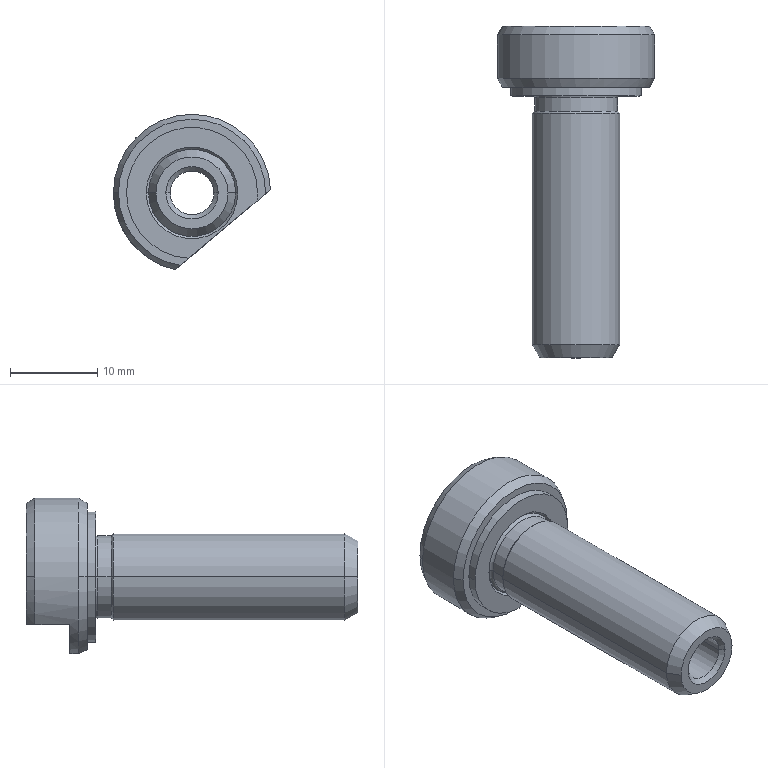Component | SolidWorks | JB_T8045.3-1999QuickChangeDrillBushing10_5_30-1 | 1 solid | 35 faces | box 17.99 x 38 x 17.79 mm | volume 3154 mm3 | cone 16 | cylinder 10 | plane 7 | torus 2 | commonest cylinder face diameters 15 x3 5 x2 10 x2 9.5 x2 18 x1 | material Nickel
STEP:
#1=COLOUR_RGB('',0.7922,0.8196,0.9333);
#2=FILL_AREA_STYLE_COLOUR('',#1);
#3=FILL_AREA_STYLE('',(#2));
#4=SURFACE_STYLE_FILL_AREA(#3);
#5=SURFACE_SIDE_STYLE('',(#4));
#6=SURFACE_STYLE_USAGE(.BOTH.,#5);
#7=PRESENTATION_STYLE_ASSIGNMENT((#6));
#8=CARTESIAN_POINT('',(-0.1628,10.827,2.067));
#9=VERTEX_POINT('',#8);
#10=CARTESIAN_POINT('',(0.1628,10.827,2.067));
#11=VERTEX_POINT('',#10);
#12=CARTESIAN_POINT('',(0.,10.827,2.067));
#13=DIRECTION('',(0.,-1.,0.));
#14=DIRECTION('',(1.,0.,0.));
#15=AXIS2_PLACEMENT_3D('',#12,#13,#14);
#16=CIRCLE('',#15,0.1628);
#17=EDGE_CURVE('',#9,#11,#16,.T.);
#18=ORIENTED_EDGE('',*,*,#17,.F.);
#19=CARTESIAN_POINT('',(-0.1969,10.886,2.067));
#20=VERTEX_POINT('',#19);
#21=CARTESIAN_POINT('',(-0.1969,10.886,2.067));
#22=DIRECTION('',(-0.5,0.866,-0.));
#23=VECTOR('',#22,39.37);
#24=LINE('',#21,#23);
#25=EDGE_CURVE('',#9,#20,#24,.T.);
#26=ORIENTED_EDGE('',*,*,#25,.T.);
#27=CARTESIAN_POINT('',(0.1969,10.886,2.067));
#28=VERTEX_POINT('',#27);
#29=CARTESIAN_POINT('',(0.,10.886,2.067));
#30=DIRECTION('',(0.,1.,0.));
#31=DIRECTION('',(1.,0.,0.));
#32=AXIS2_PLACEMENT_3D('',#29,#30,#31);
#33=CIRCLE('',#32,0.1969);
#34=EDGE_CURVE('',#28,#20,#33,.T.);
#35=ORIENTED_EDGE('',*,*,#34,.F.);
#36=CARTESIAN_POINT('',(0.1969,10.886,2.067));
#37=DIRECTION('',(0.5,0.866,0.));
#38=VECTOR('',#37,39.37);
#39=LINE('',#36,#38);
#40=EDGE_CURVE('',#11,#28,#39,.T.);
#41=ORIENTED_EDGE('',*,*,#40,.F.);
#42=EDGE_LOOP('',(#18,#26,#35,#41));
#43=FACE_OUTER_BOUND('',#42,.T.);
#44=CARTESIAN_POINT('',(0.,10.886,2.067));
#45=DIRECTION('',(0.,1.,0.));
#46=DIRECTION('',(1.,0.,0.));
#47=AXIS2_PLACEMENT_3D('',#44,#45,#46);
#48=CONICAL_SURFACE('',#47,0.1969,0.5236);
#49=ADVANCED_FACE('',(#43),#48,.T.);
#50=CARTESIAN_POINT('',(-0.1969,12.018,2.067));
#51=VERTEX_POINT('',#50);
#52=CARTESIAN_POINT('',(0.1969,12.018,2.067));
#53=VERTEX_POINT('',#52);
#54=CARTESIAN_POINT('',(0.,12.018,2.067));
#55=DIRECTION('',(0.,1.,0.));
#56=DIRECTION('',(1.,0.,0.));
#57=AXIS2_PLACEMENT_3D('',#54,#55,#56);
#58=CIRCLE('',#57,0.1969);
#59=EDGE_CURVE('',#51,#53,#58,.T.);
#60=ORIENTED_EDGE('',*,*,#59,.F.);
#61=CARTESIAN_POINT('',(-0.187,12.001,2.067));
#62=VERTEX_POINT('',#61);
#63=CARTESIAN_POINT('',(-0.2067,12.001,2.067));
#64=DIRECTION('',(0.,0.,-1.));
#65=DIRECTION('',(-1.,0.,0.));
#66=AXIS2_PLACEMENT_3D('',#63,#64,#65);
#67=CIRCLE('',#66,0.01969);
#68=EDGE_CURVE('',#51,#62,#67,.T.);
#69=ORIENTED_EDGE('',*,*,#68,.T.);
#70=CARTESIAN_POINT('',(0.187,12.001,2.067));
#71=VERTEX_POINT('',#70);
#72=CARTESIAN_POINT('',(0.,12.001,2.067));
#73=DIRECTION('',(0.,-1.,0.));
#74=DIRECTION('',(1.,0.,0.));
#75=AXIS2_PLACEMENT_3D('',#72,#73,#74);
#76=CIRCLE('',#75,0.187);
#77=EDGE_CURVE('',#71,#62,#76,.T.);
#78=ORIENTED_EDGE('',*,*,#77,.F.);
#79=CARTESIAN_POINT('',(0.2067,12.001,2.067));
#80=DIRECTION('',(-0.,0.,1.));
#81=DIRECTION('',(1.,0.,0.));
#82=AXIS2_PLACEMENT_3D('',#79,#80,#81);
#83=CIRCLE('',#82,0.01969);
#84=EDGE_CURVE('',#53,#71,#83,.T.);
#85=ORIENTED_EDGE('',*,*,#84,.F.);
#86=EDGE_LOOP('',(#60,#69,#78,#85));
#87=FACE_OUTER_BOUND('',#86,.T.);
#88=CARTESIAN_POINT('',(0.,12.001,2.067));
#89=DIRECTION('',(0.,1.,0.));
#90=DIRECTION('',(1.,0.,0.));
#91=AXIS2_PLACEMENT_3D('',#88,#89,#90);
#92=TOROIDAL_SURFACE('',#91,0.2067,0.01969);
#93=ADVANCED_FACE('',(#87),#92,.F.);
#94=ORIENTED_EDGE('',*,*,#59,.T.);
#95=CARTESIAN_POINT('',(0.2067,12.008,2.067));
#96=VERTEX_POINT('',#95);
#97=CARTESIAN_POINT('',(0.2067,12.008,2.067));
#98=DIRECTION('',(0.7071,-0.7071,0.));
#99=VECTOR('',#98,39.37);
#100=LINE('',#97,#99);
#101=EDGE_CURVE('',#53,#96,#100,.T.);
#102=ORIENTED_EDGE('',*,*,#101,.T.);
#103=CARTESIAN_POINT('',(-0.2067,12.008,2.067));
#104=VERTEX_POINT('',#103);
#105=CARTESIAN_POINT('',(0.,12.008,2.067));
#106=DIRECTION('',(0.,1.,0.));
#107=DIRECTION('',(1.,0.,0.));
#108=AXIS2_PLACEMENT_3D('',#105,#106,#107);
#109=CIRCLE('',#108,0.2067);
#110=EDGE_CURVE('',#104,#96,#109,.T.);
#111=ORIENTED_EDGE('',*,*,#110,.F.);
#112=CARTESIAN_POINT('',(-0.2067,12.008,2.067));
#113=DIRECTION('',(-0.7071,-0.7071,-0.));
#114=VECTOR('',#113,39.37);
#115=LINE('',#112,#114);
#116=EDGE_CURVE('',#51,#104,#115,.T.);
#117=ORIENTED_EDGE('',*,*,#116,.F.);
#118=EDGE_LOOP('',(#94,#102,#111,#117));
#119=FACE_OUTER_BOUND('',#118,.T.);
#120=CARTESIAN_POINT('',(0.,12.008,2.067));
#121=DIRECTION('',(0.,-1.,0.));
#122=DIRECTION('',(-1.,0.,0.));
#123=AXIS2_PLACEMENT_3D('',#120,#121,#122);
#124=CONICAL_SURFACE('',#123,0.2067,0.7854);
#125=ADVANCED_FACE('',(#119),#124,.F.);
#126=CARTESIAN_POINT('',(0.187,11.939,2.067));
#127=VERTEX_POINT('',#126);
#128=CARTESIAN_POINT('',(-0.187,11.939,2.067));
#129=VERTEX_POINT('',#128);
#130=CARTESIAN_POINT('',(0.,11.939,2.067));
#131=DIRECTION('',(0.,1.,0.));
#132=DIRECTION('',(1.,0.,0.));
#133=AXIS2_PLACEMENT_3D('',#130,#131,#132);
#134=CIRCLE('',#133,0.187);
#135=EDGE_CURVE('',#127,#129,#134,.T.);
#136=ORIENTED_EDGE('',*,*,#135,.F.);
#137=CARTESIAN_POINT('',(0.1969,11.929,2.067));
#138=VERTEX_POINT('',#137);
#139=CARTESIAN_POINT('',(0.187,11.939,2.067));
#140=DIRECTION('',(0.7071,-0.7071,0.));
#141=VECTOR('',#140,39.37);
#142=LINE('',#139,#141);
#143=EDGE_CURVE('',#127,#138,#142,.T.);
#144=ORIENTED_EDGE('',*,*,#143,.T.);
#145=CARTESIAN_POINT('',(-0.1969,11.929,2.067));
#146=VERTEX_POINT('',#145);
#147=CARTESIAN_POINT('',(0.,11.929,2.067));
#148=DIRECTION('',(0.,-1.,0.));
#149=DIRECTION('',(-1.,0.,0.));
#150=AXIS2_PLACEMENT_3D('',#147,#148,#149);
#151=CIRCLE('',#150,0.1969);
#152=EDGE_CURVE('',#146,#138,#151,.T.);
#153=ORIENTED_EDGE('',*,*,#152,.F.);
#154=CARTESIAN_POINT('',(-0.187,11.939,2.067));
#155=DIRECTION('',(-0.7071,-0.7071,-0.));
#156=VECTOR('',#155,39.37);
#157=LINE('',#154,#156);
#158=EDGE_CURVE('',#129,#146,#157,.T.);
#159=ORIENTED_EDGE('',*,*,#158,.F.);
#160=EDGE_LOOP('',(#136,#144,#153,#159));
#161=FACE_OUTER_BOUND('',#160,.T.);
#162=CARTESIAN_POINT('',(0.,11.939,2.067));
#163=DIRECTION('',(0.,-1.,0.));
#164=DIRECTION('',(-1.,0.,0.));
#165=AXIS2_PLACEMENT_3D('',#162,#163,#164);
#166=CONICAL_SURFACE('',#165,0.187,0.7854);
#167=ADVANCED_FACE('',(#161),#166,.T.);
#168=CARTESIAN_POINT('',(0.09843,10.846,2.067));
#169=VERTEX_POINT('',#168);
#170=CARTESIAN_POINT('',(-0.09843,10.846,2.067));
#171=VERTEX_POINT('',#170);
#172=CARTESIAN_POINT('',(0.,10.846,2.067));
#173=DIRECTION('',(0.,-1.,0.));
#174=DIRECTION('',(1.,0.,0.));
#175=AXIS2_PLACEMENT_3D('',#172,#173,#174);
#176=CIRCLE('',#175,0.09843);
#177=EDGE_CURVE('',#169,#171,#176,.T.);
#178=ORIENTED_EDGE('',*,*,#177,.F.);
#179=CARTESIAN_POINT('',(0.1181,10.827,2.067));
#180=VERTEX_POINT('',#179);
#181=CARTESIAN_POINT('',(0.1181,10.827,2.067));
#182=DIRECTION('',(0.7071,-0.7071,0.));
#183=VECTOR('',#182,39.37);
#184=LINE('',#181,#183);
#185=EDGE_CURVE('',#169,#180,#184,.T.);
#186=ORIENTED_EDGE('',*,*,#185,.T.);
#187=CARTESIAN_POINT('',(-0.1181,10.827,2.067));
#188=VERTEX_POINT('',#187);
#189=CARTESIAN_POINT('',(0.,10.827,2.067));
#190=DIRECTION('',(0.,1.,0.));
#191=DIRECTION('',(1.,0.,0.));
#192=AXIS2_PLACEMENT_3D('',#189,#190,#191);
#193=CIRCLE('',#192,0.1181);
#194=EDGE_CURVE('',#188,#180,#193,.T.);
#195=ORIENTED_EDGE('',*,*,#194,.F.);
#196=CARTESIAN_POINT('',(-0.1181,10.827,2.067));
#197=DIRECTION('',(-0.7071,-0.7071,-0.));
#198=VECTOR('',#197,39.37);
#199=LINE('',#196,#198);
#200=EDGE_CURVE('',#171,#188,#199,.T.);
#201=ORIENTED_EDGE('',*,*,#200,.F.);
#202=EDGE_LOOP('',(#178,#186,#195,#201));
#203=FACE_OUTER_BOUND('',#202,.T.);
#204=CARTESIAN_POINT('',(0.,10.827,2.067));
#205=DIRECTION('',(0.,-1.,0.));
#206=DIRECTION('',(-1.,0.,0.));
#207=AXIS2_PLACEMENT_3D('',#204,#205,#206);
#208=CONICAL_SURFACE('',#207,0.1181,0.7854);
#209=ADVANCED_FACE('',(#203),#208,.F.);
#210=CARTESIAN_POINT('',(-0.09843,12.264,2.067));
#211=VERTEX_POINT('',#210);
#212=CARTESIAN_POINT('',(0.09843,12.264,2.067));
#213=VERTEX_POINT('',#212);
#214=CARTESIAN_POINT('',(0.,12.264,2.067));
#215=DIRECTION('',(0.,1.,0.));
#216=DIRECTION('',(-1.,0.,0.));
#217=AXIS2_PLACEMENT_3D('',#214,#215,#216);
#218=CIRCLE('',#217,0.09843);
#219=EDGE_CURVE('',#211,#213,#218,.T.);
#220=ORIENTED_EDGE('',*,*,#219,.F.);
#221=CARTESIAN_POINT('',(-0.1325,12.323,2.067));
#222=VERTEX_POINT('',#221);
#223=CARTESIAN_POINT('',(-0.09843,12.264,2.067));
#224=DIRECTION('',(-0.5,0.866,-0.));
#225=VECTOR('',#224,39.37);
#226=LINE('',#223,#225);
#227=EDGE_CURVE('',#211,#222,#226,.T.);
#228=ORIENTED_EDGE('',*,*,#227,.T.);
#229=CARTESIAN_POINT('',(0.1325,12.323,2.067));
#230=VERTEX_POINT('',#229);
#231=CARTESIAN_POINT('',(0.,12.323,2.067));
#232=DIRECTION('',(0.,-1.,0.));
#233=DIRECTION('',(-1.,0.,0.));
#234=AXIS2_PLACEMENT_3D('',#231,#232,#233);
#235=CIRCLE('',#234,0.1325);
#236=EDGE_CURVE('',#230,#222,#235,.T.);
#237=ORIENTED_EDGE('',*,*,#236,.F.);
#238=CARTESIAN_POINT('',(0.09843,12.264,2.067));
#239=DIRECTION('',(0.5,0.866,0.));
#240=VECTOR('',#239,39.37);
#241=LINE('',#238,#240);
#242=EDGE_CURVE('',#213,#230,#241,.T.);
#243=ORIENTED_EDGE('',*,*,#242,.F.);
#244=EDGE_LOOP('',(#220,#228,#237,#243));
#245=FACE_OUTER_BOUND('',#244,.T.);
#246=CARTESIAN_POINT('',(0.,12.264,2.067));
#247=DIRECTION('',(0.,1.,0.));
#248=DIRECTION('',(1.,0.,0.));
#249=AXIS2_PLACEMENT_3D('',#246,#247,#248);
#250=CONICAL_SURFACE('',#249,0.09843,0.5236);
#251=ADVANCED_FACE('',(#245),#250,.F.);
#252=ORIENTED_EDGE('',*,*,#177,.T.);
#253=CARTESIAN_POINT('',(-0.09843,16.352,2.067));
#254=DIRECTION('',(0.,1.,0.));
#255=VECTOR('',#254,39.37);
#256=LINE('',#253,#255);
#257=EDGE_CURVE('',#171,#211,#256,.T.);
#258=ORIENTED_EDGE('',*,*,#257,.T.);
#259=ORIENTED_EDGE('',*,*,#219,.T.);
#260=CARTESIAN_POINT('',(0.09843,16.352,2.067));
#261=DIRECTION('',(0.,1.,0.));
#262=VECTOR('',#261,39.37);
#263=LINE('',#260,#262);
#264=EDGE_CURVE('',#169,#213,#263,.T.);
#265=ORIENTED_EDGE('',*,*,#264,.F.);
#266=EDGE_LOOP('',(#252,#258,#259,#265));
#267=FACE_OUTER_BOUND('',#266,.T.);
#268=CARTESIAN_POINT('',(0.,16.352,2.067));
#269=DIRECTION('',(0.,1.,0.));
#270=DIRECTION('',(1.,0.,0.));
#271=AXIS2_PLACEMENT_3D('',#268,#269,#270);
#272=CYLINDRICAL_SURFACE('',#271,0.09843);
#273=ADVANCED_FACE('',(#267),#272,.F.);
#274=ORIENTED_EDGE('',*,*,#34,.T.);
#275=CARTESIAN_POINT('',(-0.1969,16.352,2.067));
#276=DIRECTION('',(0.,1.,0.));
#277=VECTOR('',#276,39.37);
#278=LINE('',#275,#277);
#279=EDGE_CURVE('',#20,#146,#278,.T.);
#280=ORIENTED_EDGE('',*,*,#279,.T.);
#281=ORIENTED_EDGE('',*,*,#152,.T.);
#282=CARTESIAN_POINT('',(0.1969,16.352,2.067));
#283=DIRECTION('',(0.,1.,0.));
#284=VECTOR('',#283,39.37);
#285=LINE('',#282,#284);
#286=EDGE_CURVE('',#28,#138,#285,.T.);
#287=ORIENTED_EDGE('',*,*,#286,.F.);
#288=EDGE_LOOP('',(#274,#280,#281,#287));
#289=FACE_OUTER_BOUND('',#288,.T.);
#290=CARTESIAN_POINT('',(0.,16.352,2.067));
#291=DIRECTION('',(0.,1.,0.));
#292=DIRECTION('',(1.,0.,0.));
#293=AXIS2_PLACEMENT_3D('',#290,#291,#292);
#294=CYLINDRICAL_SURFACE('',#293,0.1969);
#295=ADVANCED_FACE('',(#289),#294,.T.);
#296=ORIENTED_EDGE('',*,*,#135,.T.);
#297=CARTESIAN_POINT('',(-0.187,16.352,2.067));
#298=DIRECTION('',(0.,1.,0.));
#299=VECTOR('',#298,39.37);
#300=LINE('',#297,#299);
#301=EDGE_CURVE('',#129,#62,#300,.T.);
#302=ORIENTED_EDGE('',*,*,#301,.T.);
#303=CARTESIAN_POINT('',(0.,12.001,2.067));
#304=DIRECTION('',(0.,-1.,0.));
#305=DIRECTION('',(1.,0.,0.));
#306=AXIS2_PLACEMENT_3D('',#303,#304,#305);
#307=CIRCLE('',#306,0.187);
#308=EDGE_CURVE('',#62,#71,#307,.T.);
#309=ORIENTED_EDGE('',*,*,#308,.T.);
#310=CARTESIAN_POINT('',(0.187,16.352,2.067));
#311=DIRECTION('',(0.,1.,0.));
#312=VECTOR('',#311,39.37);
#313=LINE('',#310,#312);
#314=EDGE_CURVE('',#127,#71,#313,.T.);
#315=ORIENTED_EDGE('',*,*,#314,.F.);
#316=EDGE_LOOP('',(#296,#302,#309,#315));
#317=FACE_OUTER_BOUND('',#316,.T.);
#318=CARTESIAN_POINT('',(0.,16.352,2.067));
#319=DIRECTION('',(0.,1.,0.));
#320=DIRECTION('',(1.,0.,0.));
#321=AXIS2_PLACEMENT_3D('',#318,#319,#320);
#322=CYLINDRICAL_SURFACE('',#321,0.187);
#323=ADVANCED_FACE('',(#317),#322,.T.);
#324=CARTESIAN_POINT('',(-0.3316,12.047,2.067));
#325=VERTEX_POINT('',#324);
#326=CARTESIAN_POINT('',(-0.0532,12.047,1.74));
#327=VERTEX_POINT('',#326);
#328=CARTESIAN_POINT('',(0.,12.047,2.067));
#329=DIRECTION('',(0.,-1.,0.));
#330=DIRECTION('',(1.,0.,-0.));
#331=AXIS2_PLACEMENT_3D('',#328,#329,#330);
#332=CIRCLE('',#331,0.3316);
#333=EDGE_CURVE('',#325,#327,#332,.T.);
#334=ORIENTED_EDGE('',*,*,#333,.F.);
#335=CARTESIAN_POINT('',(-0.3543,12.087,2.067));
#336=VERTEX_POINT('',#335);
#337=CARTESIAN_POINT('',(-0.3543,12.087,2.067));
#338=DIRECTION('',(-0.5,0.866,-0.));
#339=VECTOR('',#338,39.37);
#340=LINE('',#337,#339);
#341=EDGE_CURVE('',#325,#336,#340,.T.);
#342=ORIENTED_EDGE('',*,*,#341,.T.);
#343=CARTESIAN_POINT('',(-0.07566,12.087,1.721));
#344=VERTEX_POINT('',#343);
#345=CARTESIAN_POINT('',(0.,12.087,2.067));
#346=DIRECTION('',(0.,1.,0.));
#347=DIRECTION('',(1.,0.,0.));
#348=AXIS2_PLACEMENT_3D('',#345,#346,#347);
#349=CIRCLE('',#348,0.3543);
#350=EDGE_CURVE('',#344,#336,#349,.T.);
#351=ORIENTED_EDGE('',*,*,#350,.F.);
#352=CARTESIAN_POINT('',(-0.07566,12.087,1.721));
#353=CARTESIAN_POINT('',(-0.06828,12.073,1.727));
#354=CARTESIAN_POINT('',(-0.0608,12.06,1.733));
#355=CARTESIAN_POINT('',(-0.0532,12.047,1.74));
#356=B_SPLINE_CURVE_WITH_KNOTS('',3,(#352,#353,#354,#355),.UNSPECIFIED.,.F.,.F.,(4,4),(0.01817,0.01941),.UNSPECIFIED.);
#357=EDGE_CURVE('',#344,#327,#356,.T.);
#358=ORIENTED_EDGE('',*,*,#357,.T.);
#359=EDGE_LOOP('',(#334,#342,#351,#358));
#360=FACE_OUTER_BOUND('',#359,.T.);
#361=CARTESIAN_POINT('',(0.,12.087,2.067));
#362=DIRECTION('',(0.,1.,0.));
#363=DIRECTION('',(1.,0.,0.));
#364=AXIS2_PLACEMENT_3D('',#361,#362,#363);
#365=CONICAL_SURFACE('',#364,0.3543,0.5236);
#366=ADVANCED_FACE('',(#360),#365,.T.);
#367=ORIENTED_EDGE('',*,*,#341,.F.);
#368=CARTESIAN_POINT('',(0.3316,12.047,2.067));
#369=VERTEX_POINT('',#368);
#370=CARTESIAN_POINT('',(0.,12.047,2.067));
#371=DIRECTION('',(0.,-1.,0.));
#372=DIRECTION('',(1.,0.,0.));
#373=AXIS2_PLACEMENT_3D('',#370,#371,#372);
#374=CIRCLE('',#373,0.3316);
#375=EDGE_CURVE('',#369,#325,#374,.T.);
#376=ORIENTED_EDGE('',*,*,#375,.F.);
#377=CARTESIAN_POINT('',(0.3369,12.056,2.067));
#378=VERTEX_POINT('',#377);
#379=CARTESIAN_POINT('',(0.3543,12.087,2.067));
#380=DIRECTION('',(0.5,0.866,0.));
#381=VECTOR('',#380,39.37);
#382=LINE('',#379,#381);
#383=EDGE_CURVE('',#369,#378,#382,.T.);
#384=ORIENTED_EDGE('',*,*,#383,.T.);
#385=CARTESIAN_POINT('',(0.354,12.087,2.081));
#386=VERTEX_POINT('',#385);
#387=CARTESIAN_POINT('',(0.3369,12.056,2.067));
#388=CARTESIAN_POINT('',(0.3427,12.066,2.072));
#389=CARTESIAN_POINT('',(0.3484,12.076,2.077));
#390=CARTESIAN_POINT('',(0.354,12.087,2.081));
#391=B_SPLINE_CURVE_WITH_KNOTS('',3,(#387,#388,#389,#390),.UNSPECIFIED.,.F.,.F.,(4,4),(0.03623,0.03717),.UNSPECIFIED.);
#392=EDGE_CURVE('',#378,#386,#391,.T.);
#393=ORIENTED_EDGE('',*,*,#392,.T.);
#394=CARTESIAN_POINT('',(0.,12.087,2.067));
#395=DIRECTION('',(0.,1.,0.));
#396=DIRECTION('',(1.,0.,0.));
#397=AXIS2_PLACEMENT_3D('',#394,#395,#396);
#398=CIRCLE('',#397,0.3543);
#399=EDGE_CURVE('',#336,#386,#398,.T.);
#400=ORIENTED_EDGE('',*,*,#399,.F.);
#401=EDGE_LOOP('',(#367,#376,#384,#393,#400));
#402=FACE_OUTER_BOUND('',#401,.T.);
#403=CARTESIAN_POINT('',(0.,12.087,2.067));
#404=DIRECTION('',(0.,1.,0.));
#405=DIRECTION('',(1.,0.,0.));
#406=AXIS2_PLACEMENT_3D('',#403,#404,#405);
#407=CONICAL_SURFACE('',#406,0.3543,0.5236);
#408=ADVANCED_FACE('',(#402),#407,.T.);
#409=CARTESIAN_POINT('',(-0.01459,12.008,1.772));
#410=VERTEX_POINT('',#409);
#411=CARTESIAN_POINT('',(-0.2953,12.008,2.067));
#412=VERTEX_POINT('',#411);
#413=CARTESIAN_POINT('',(0.,12.008,2.067));
#414=DIRECTION('',(0.,1.,0.));
#415=DIRECTION('',(1.,0.,0.));
#416=AXIS2_PLACEMENT_3D('',#413,#414,#415);
#417=CIRCLE('',#416,0.2953);
#418=EDGE_CURVE('',#410,#412,#417,.T.);
#419=ORIENTED_EDGE('',*,*,#418,.T.);
#420=CARTESIAN_POINT('',(-0.2953,12.047,2.067));
#421=VERTEX_POINT('',#420);
#422=CARTESIAN_POINT('',(-0.2953,16.352,2.067));
#423=DIRECTION('',(0.,1.,0.));
#424=VECTOR('',#423,39.37);
#425=LINE('',#422,#424);
#426=EDGE_CURVE('',#412,#421,#425,.T.);
#427=ORIENTED_EDGE('',*,*,#426,.T.);
#428=CARTESIAN_POINT('',(-0.01459,12.047,1.772));
#429=VERTEX_POINT('',#428);
#430=CARTESIAN_POINT('',(0.,12.047,2.067));
#431=DIRECTION('',(0.,1.,0.));
#432=DIRECTION('',(1.,0.,0.));
#433=AXIS2_PLACEMENT_3D('',#430,#431,#432);
#434=CIRCLE('',#433,0.2953);
#435=EDGE_CURVE('',#429,#421,#434,.T.);
#436=ORIENTED_EDGE('',*,*,#435,.F.);
#437=CARTESIAN_POINT('',(-0.01459,16.352,1.772));
#438=DIRECTION('',(0.,1.,0.));
#439=VECTOR('',#438,39.37);
#440=LINE('',#437,#439);
#441=EDGE_CURVE('',#410,#429,#440,.T.);
#442=ORIENTED_EDGE('',*,*,#441,.F.);
#443=EDGE_LOOP('',(#419,#427,#436,#442));
#444=FACE_OUTER_BOUND('',#443,.T.);
#445=CARTESIAN_POINT('',(0.,16.352,2.067));
#446=DIRECTION('',(0.,1.,0.));
#447=DIRECTION('',(1.,0.,0.));
#448=AXIS2_PLACEMENT_3D('',#445,#446,#447);
#449=CYLINDRICAL_SURFACE('',#448,0.2953);
#450=ADVANCED_FACE('',(#444),#449,.T.);
#451=ORIENTED_EDGE('',*,*,#426,.F.);
#452=CARTESIAN_POINT('',(0.2953,12.008,2.067));
#453=VERTEX_POINT('',#452);
#454=CARTESIAN_POINT('',(0.,12.008,2.067));
#455=DIRECTION('',(0.,1.,0.));
#456=DIRECTION('',(1.,0.,0.));
#457=AXIS2_PLACEMENT_3D('',#454,#455,#456);
#458=CIRCLE('',#457,0.2953);
#459=EDGE_CURVE('',#412,#453,#458,.T.);
#460=ORIENTED_EDGE('',*,*,#459,.T.);
#461=CARTESIAN_POINT('',(0.2953,12.047,2.067));
#462=VERTEX_POINT('',#461);
#463=CARTESIAN_POINT('',(0.2953,16.352,2.067));
#464=DIRECTION('',(0.,1.,0.));
#465=VECTOR('',#464,39.37);
#466=LINE('',#463,#465);
#467=EDGE_CURVE('',#453,#462,#466,.T.);
#468=ORIENTED_EDGE('',*,*,#467,.T.);
#469=CARTESIAN_POINT('',(0.,12.047,2.067));
#470=DIRECTION('',(0.,1.,0.));
#471=DIRECTION('',(1.,0.,0.));
#472=AXIS2_PLACEMENT_3D('',#469,#470,#471);
#473=CIRCLE('',#472,0.2953);
#474=EDGE_CURVE('',#421,#462,#473,.T.);
#475=ORIENTED_EDGE('',*,*,#474,.F.);
#476=EDGE_LOOP('',(#451,#460,#468,#475));
#477=FACE_OUTER_BOUND('',#476,.T.);
#478=CARTESIAN_POINT('',(0.,16.352,2.067));
#479=DIRECTION('',(0.,1.,0.));
#480=DIRECTION('',(1.,0.,0.));
#481=AXIS2_PLACEMENT_3D('',#478,#479,#480);
#482=CYLINDRICAL_SURFACE('',#481,0.2953);
#483=ADVANCED_FACE('',(#477),#482,.T.);
#484=CARTESIAN_POINT('',(0.3316,12.323,2.067));
#485=VERTEX_POINT('',#484);
#486=CARTESIAN_POINT('',(0.3316,12.323,2.062));
#487=VERTEX_POINT('',#486);
#488=CARTESIAN_POINT('',(0.,12.323,2.067));
#489=DIRECTION('',(0.,1.,0.));
#490=DIRECTION('',(-1.,0.,0.));
#491=AXIS2_PLACEMENT_3D('',#488,#489,#490);
#492=CIRCLE('',#491,0.3316);
#493=EDGE_CURVE('',#485,#487,#492,.T.);
#494=ORIENTED_EDGE('',*,*,#493,.F.);
#495=CARTESIAN_POINT('',(0.3369,12.314,2.067));
#496=VERTEX_POINT('',#495);
#497=CARTESIAN_POINT('',(0.3316,12.323,2.067));
#498=DIRECTION('',(0.5,-0.866,0.));
#499=VECTOR('',#498,39.37);
#500=LINE('',#497,#499);
#501=EDGE_CURVE('',#485,#496,#500,.T.);
#502=ORIENTED_EDGE('',*,*,#501,.T.);
#503=CARTESIAN_POINT('',(0.3369,12.314,2.067));
#504=CARTESIAN_POINT('',(0.3351,12.317,2.065));
#505=CARTESIAN_POINT('',(0.3333,12.32,2.064));
#506=CARTESIAN_POINT('',(0.3316,12.323,2.062));
#507=B_SPLINE_CURVE_WITH_KNOTS('',3,(#503,#504,#505,#506),.UNSPECIFIED.,.F.,.F.,(4,4),(0.01747,0.01777),.UNSPECIFIED.);
#508=EDGE_CURVE('',#496,#487,#507,.T.);
#509=ORIENTED_EDGE('',*,*,#508,.T.);
#510=EDGE_LOOP('',(#494,#502,#509));
#511=FACE_OUTER_BOUND('',#510,.T.);
#512=CARTESIAN_POINT('',(0.,12.323,2.067));
#513=DIRECTION('',(0.,-1.,0.));
#514=DIRECTION('',(-1.,0.,0.));
#515=AXIS2_PLACEMENT_3D('',#512,#513,#514);
#516=CONICAL_SURFACE('',#515,0.3316,0.5236);
#517=ADVANCED_FACE('',(#511),#516,.T.);
#518=ORIENTED_EDGE('',*,*,#501,.F.);
#519=CARTESIAN_POINT('',(-0.3316,12.323,2.067));
#520=VERTEX_POINT('',#519);
#521=CARTESIAN_POINT('',(0.,12.323,2.067));
#522=DIRECTION('',(0.,1.,0.));
#523=DIRECTION('',(-1.,0.,0.));
#524=AXIS2_PLACEMENT_3D('',#521,#522,#523);
#525=CIRCLE('',#524,0.3316);
#526=EDGE_CURVE('',#520,#485,#525,.T.);
#527=ORIENTED_EDGE('',*,*,#526,.F.);
#528=CARTESIAN_POINT('',(-0.3543,12.283,2.067));
#529=VERTEX_POINT('',#528);
#530=CARTESIAN_POINT('',(-0.3316,12.323,2.067));
#531=DIRECTION('',(-0.5,-0.866,-0.));
#532=VECTOR('',#531,39.37);
#533=LINE('',#530,#532);
#534=EDGE_CURVE('',#520,#529,#533,.T.);
#535=ORIENTED_EDGE('',*,*,#534,.T.);
#536=CARTESIAN_POINT('',(0.354,12.283,2.081));
#537=VERTEX_POINT('',#536);
#538=CARTESIAN_POINT('',(0.,12.283,2.067));
#539=DIRECTION('',(0.,-1.,0.));
#540=DIRECTION('',(-1.,0.,0.));
#541=AXIS2_PLACEMENT_3D('',#538,#539,#540);
#542=CIRCLE('',#541,0.3543);
#543=EDGE_CURVE('',#537,#529,#542,.T.);
#544=ORIENTED_EDGE('',*,*,#543,.F.);
#545=CARTESIAN_POINT('',(0.354,12.283,2.081));
#546=CARTESIAN_POINT('',(0.3484,12.294,2.077));
#547=CARTESIAN_POINT('',(0.3427,12.304,2.072));
#548=CARTESIAN_POINT('',(0.3369,12.314,2.067));
#549=B_SPLINE_CURVE_WITH_KNOTS('',3,(#545,#546,#547,#548),.UNSPECIFIED.,.F.,.F.,(4,4),(0.01652,0.01747),.UNSPECIFIED.);
#550=EDGE_CURVE('',#537,#496,#549,.T.);
#551=ORIENTED_EDGE('',*,*,#550,.T.);
#552=EDGE_LOOP('',(#518,#527,#535,#544,#551));
#553=FACE_OUTER_BOUND('',#552,.T.);
#554=CARTESIAN_POINT('',(0.,12.323,2.067));
#555=DIRECTION('',(0.,-1.,0.));
#556=DIRECTION('',(-1.,0.,0.));
#557=AXIS2_PLACEMENT_3D('',#554,#555,#556);
#558=CONICAL_SURFACE('',#557,0.3316,0.5236);
#559=ADVANCED_FACE('',(#553),#558,.T.);
#560=CARTESIAN_POINT('',(-0.07566,12.126,1.721));
#561=VERTEX_POINT('',#560);
#562=CARTESIAN_POINT('',(-0.07566,16.352,1.721));
#563=DIRECTION('',(0.,1.,0.));
#564=VECTOR('',#563,39.37);
#565=LINE('',#562,#564);
#566=EDGE_CURVE('',#344,#561,#565,.T.);
#567=ORIENTED_EDGE('',*,*,#566,.F.);
#568=ORIENTED_EDGE('',*,*,#350,.T.);
#569=ORIENTED_EDGE('',*,*,#399,.T.);
#570=CARTESIAN_POINT('',(0.354,16.352,2.081));
#571=DIRECTION('',(0.,-1.,0.));
#572=VECTOR('',#571,39.37);
#573=LINE('',#570,#572);
#574=EDGE_CURVE('',#537,#386,#573,.T.);
#575=ORIENTED_EDGE('',*,*,#574,.F.);
#576=ORIENTED_EDGE('',*,*,#543,.T.);
#577=CARTESIAN_POINT('',(-0.2805,12.283,1.85));
#578=VERTEX_POINT('',#577);
#579=CARTESIAN_POINT('',(0.,12.283,2.067));
#580=DIRECTION('',(0.,-1.,0.));
#581=DIRECTION('',(-1.,0.,0.));
#582=AXIS2_PLACEMENT_3D('',#579,#580,#581);
#583=CIRCLE('',#582,0.3543);
#584=EDGE_CURVE('',#529,#578,#583,.T.);
#585=ORIENTED_EDGE('',*,*,#584,.T.);
#586=CARTESIAN_POINT('',(-0.2805,12.126,1.85));
#587=VERTEX_POINT('',#586);
#588=CARTESIAN_POINT('',(-0.2805,16.352,1.85));
#589=DIRECTION('',(0.,1.,0.));
#590=VECTOR('',#589,39.37);
#591=LINE('',#588,#590);
#592=EDGE_CURVE('',#587,#578,#591,.T.);
#593=ORIENTED_EDGE('',*,*,#592,.F.);
#594=CARTESIAN_POINT('',(0.,12.126,2.067));
#595=DIRECTION('',(0.,1.,0.));
#596=DIRECTION('',(1.,0.,0.));
#597=AXIS2_PLACEMENT_3D('',#594,#595,#596);
#598=CIRCLE('',#597,0.3543);
#599=EDGE_CURVE('',#561,#587,#598,.T.);
#600=ORIENTED_EDGE('',*,*,#599,.F.);
#601=EDGE_LOOP('',(#567,#568,#569,#575,#576,#585,#593,#600));
#602=FACE_OUTER_BOUND('',#601,.T.);
#603=CARTESIAN_POINT('',(0.,16.352,2.067));
#604=DIRECTION('',(0.,1.,0.));
#605=DIRECTION('',(1.,0.,0.));
#606=AXIS2_PLACEMENT_3D('',#603,#604,#605);
#607=CYLINDRICAL_SURFACE('',#606,0.3543);
#608=ADVANCED_FACE('',(#602),#607,.T.);
#609=ORIENTED_EDGE('',*,*,#236,.T.);
#610=CARTESIAN_POINT('',(0.,12.323,2.067));
#611=DIRECTION('',(0.,-1.,0.));
#612=DIRECTION('',(-1.,0.,0.));
#613=AXIS2_PLACEMENT_3D('',#610,#611,#612);
#614=CIRCLE('',#613,0.1325);
#615=EDGE_CURVE('',#222,#230,#614,.T.);
#616=ORIENTED_EDGE('',*,*,#615,.T.);
#617=EDGE_LOOP('',(#609,#616));
#618=FACE_BOUND('',#617,.T.);
#619=CARTESIAN_POINT('',(0.07881,12.323,1.85));
#620=VERTEX_POINT('',#619);
#621=CARTESIAN_POINT('',(0.09072,12.323,1.86));
#622=DIRECTION('',(0.766,0.,0.6428));
#623=VECTOR('',#622,39.37);
#624=LINE('',#621,#623);
#625=EDGE_CURVE('',#620,#487,#624,.T.);
#626=ORIENTED_EDGE('',*,*,#625,.F.);
#627=CARTESIAN_POINT('',(-0.2511,12.323,1.85));
#628=VERTEX_POINT('',#627);
#629=CARTESIAN_POINT('',(0.,12.323,1.85));
#630=DIRECTION('',(1.,0.,0.));
#631=VECTOR('',#630,39.37);
#632=LINE('',#629,#631);
#633=EDGE_CURVE('',#628,#620,#632,.T.);
#634=ORIENTED_EDGE('',*,*,#633,.F.);
#635=CARTESIAN_POINT('',(0.,12.323,2.067));
#636=DIRECTION('',(0.,1.,0.));
#637=DIRECTION('',(-1.,0.,0.));
#638=AXIS2_PLACEMENT_3D('',#635,#636,#637);
#639=CIRCLE('',#638,0.3316);
#640=EDGE_CURVE('',#628,#520,#639,.T.);
#641=ORIENTED_EDGE('',*,*,#640,.T.);
#642=ORIENTED_EDGE('',*,*,#526,.T.);
#643=ORIENTED_EDGE('',*,*,#493,.T.);
#644=EDGE_LOOP('',(#626,#634,#641,#642,#643));
#645=FACE_OUTER_BOUND('',#644,.T.);
#646=CARTESIAN_POINT('',(0.,12.323,1.969));
#647=DIRECTION('',(0.,-1.,0.));
#648=DIRECTION('',(-1.,0.,-0.));
#649=AXIS2_PLACEMENT_3D('',#646,#647,#648);
#650=PLANE('',#649);
#651=ADVANCED_FACE('',(#618,#645),#650,.F.);
#652=ORIENTED_EDGE('',*,*,#534,.F.);
#653=ORIENTED_EDGE('',*,*,#640,.F.);
#654=CARTESIAN_POINT('',(-0.2511,12.323,1.85));
#655=CARTESIAN_POINT('',(-0.2611,12.31,1.85));
#656=CARTESIAN_POINT('',(-0.2708,12.297,1.85));
#657=CARTESIAN_POINT('',(-0.2805,12.283,1.85));
#658=B_SPLINE_CURVE_WITH_KNOTS('',3,(#654,#655,#656,#657),.UNSPECIFIED.,.F.,.F.,(4,4),(0.03099,0.03225),.UNSPECIFIED.);
#659=EDGE_CURVE('',#628,#578,#658,.T.);
#660=ORIENTED_EDGE('',*,*,#659,.T.);
#661=ORIENTED_EDGE('',*,*,#584,.F.);
#662=EDGE_LOOP('',(#652,#653,#660,#661));
#663=FACE_OUTER_BOUND('',#662,.T.);
#664=CARTESIAN_POINT('',(0.,12.323,2.067));
#665=DIRECTION('',(0.,-1.,0.));
#666=DIRECTION('',(-1.,0.,0.));
#667=AXIS2_PLACEMENT_3D('',#664,#665,#666);
#668=CONICAL_SURFACE('',#667,0.3316,0.5236);
#669=ADVANCED_FACE('',(#663),#668,.T.);
#670=CARTESIAN_POINT('',(0.3316,12.047,2.062));
#671=VERTEX_POINT('',#670);
#672=CARTESIAN_POINT('',(0.293,12.047,2.03));
#673=VERTEX_POINT('',#672);
#674=CARTESIAN_POINT('',(-0.03529,12.047,1.755));
#675=DIRECTION('',(-0.766,0.,-0.6428));
#676=VECTOR('',#675,39.37);
#677=LINE('',#674,#676);
#678=EDGE_CURVE('',#671,#673,#677,.T.);
#679=ORIENTED_EDGE('',*,*,#678,.F.);
#680=CARTESIAN_POINT('',(0.,12.047,2.067));
#681=DIRECTION('',(0.,-1.,0.));
#682=DIRECTION('',(1.,0.,0.));
#683=AXIS2_PLACEMENT_3D('',#680,#681,#682);
#684=CIRCLE('',#683,0.3316);
#685=EDGE_CURVE('',#671,#369,#684,.T.);
#686=ORIENTED_EDGE('',*,*,#685,.T.);
#687=ORIENTED_EDGE('',*,*,#375,.T.);
#688=ORIENTED_EDGE('',*,*,#333,.T.);
#689=CARTESIAN_POINT('',(-0.03529,12.047,1.755));
#690=DIRECTION('',(-0.766,0.,-0.6428));
#691=VECTOR('',#690,39.37);
#692=LINE('',#689,#691);
#693=EDGE_CURVE('',#429,#327,#692,.T.);
#694=ORIENTED_EDGE('',*,*,#693,.F.);
#695=ORIENTED_EDGE('',*,*,#435,.T.);
#696=ORIENTED_EDGE('',*,*,#474,.T.);
#697=CARTESIAN_POINT('',(0.,12.047,2.067));
#698=DIRECTION('',(0.,1.,0.));
#699=DIRECTION('',(1.,0.,0.));
#700=AXIS2_PLACEMENT_3D('',#697,#698,#699);
#701=CIRCLE('',#700,0.2953);
#702=EDGE_CURVE('',#462,#673,#701,.T.);
#703=ORIENTED_EDGE('',*,*,#702,.T.);
#704=EDGE_LOOP('',(#679,#686,#687,#688,#694,#695,#696,#703));
#705=FACE_OUTER_BOUND('',#704,.T.);
#706=CARTESIAN_POINT('',(0.,12.047,1.713));
#707=DIRECTION('',(0.,1.,0.));
#708=DIRECTION('',(1.,0.,0.));
#709=AXIS2_PLACEMENT_3D('',#706,#707,#708);
#710=PLANE('',#709);
#711=ADVANCED_FACE('',(#705),#710,.F.);
#712=ORIENTED_EDGE('',*,*,#467,.F.);
#713=CARTESIAN_POINT('',(0.293,12.008,2.03));
#714=VERTEX_POINT('',#713);
#715=CARTESIAN_POINT('',(0.,12.008,2.067));
#716=DIRECTION('',(0.,1.,0.));
#717=DIRECTION('',(1.,0.,0.));
#718=AXIS2_PLACEMENT_3D('',#715,#716,#717);
#719=CIRCLE('',#718,0.2953);
#720=EDGE_CURVE('',#453,#714,#719,.T.);
#721=ORIENTED_EDGE('',*,*,#720,.T.);
#722=CARTESIAN_POINT('',(0.293,16.352,2.03));
#723=DIRECTION('',(0.,-1.,0.));
#724=VECTOR('',#723,39.37);
#725=LINE('',#722,#724);
#726=EDGE_CURVE('',#673,#714,#725,.T.);
#727=ORIENTED_EDGE('',*,*,#726,.F.);
#728=ORIENTED_EDGE('',*,*,#702,.F.);
#729=EDGE_LOOP('',(#712,#721,#727,#728));
#730=FACE_OUTER_BOUND('',#729,.T.);
#731=CARTESIAN_POINT('',(0.,16.352,2.067));
#732=DIRECTION('',(0.,1.,0.));
#733=DIRECTION('',(1.,0.,0.));
#734=AXIS2_PLACEMENT_3D('',#731,#732,#733);
#735=CYLINDRICAL_SURFACE('',#734,0.2953);
#736=ADVANCED_FACE('',(#730),#735,.T.);
#737=ORIENTED_EDGE('',*,*,#110,.T.);
#738=CARTESIAN_POINT('',(0.,12.008,2.067));
#739=DIRECTION('',(0.,1.,0.));
#740=DIRECTION('',(1.,0.,0.));
#741=AXIS2_PLACEMENT_3D('',#738,#739,#740);
#742=CIRCLE('',#741,0.2067);
#743=EDGE_CURVE('',#96,#104,#742,.T.);
#744=ORIENTED_EDGE('',*,*,#743,.T.);
#745=EDGE_LOOP('',(#737,#744));
#746=FACE_BOUND('',#745,.T.);
#747=CARTESIAN_POINT('',(-0.006208,12.008,1.779));
#748=DIRECTION('',(-0.766,0.,-0.6428));
#749=VECTOR('',#748,39.37);
#750=LINE('',#747,#749);
#751=EDGE_CURVE('',#714,#410,#750,.T.);
#752=ORIENTED_EDGE('',*,*,#751,.F.);
#753=ORIENTED_EDGE('',*,*,#720,.F.);
#754=ORIENTED_EDGE('',*,*,#459,.F.);
#755=ORIENTED_EDGE('',*,*,#418,.F.);
#756=EDGE_LOOP('',(#752,#753,#754,#755));
#757=FACE_OUTER_BOUND('',#756,.T.);
#758=CARTESIAN_POINT('',(0.,12.008,1.772));
#759=DIRECTION('',(0.,1.,0.));
#760=DIRECTION('',(1.,0.,0.));
#761=AXIS2_PLACEMENT_3D('',#758,#759,#760);
#762=PLANE('',#761);
#763=ADVANCED_FACE('',(#746,#757),#762,.F.);
#764=ORIENTED_EDGE('',*,*,#383,.F.);
#765=ORIENTED_EDGE('',*,*,#685,.F.);
#766=CARTESIAN_POINT('',(0.3316,12.047,2.062));
#767=CARTESIAN_POINT('',(0.3333,12.05,2.064));
#768=CARTESIAN_POINT('',(0.3351,12.053,2.065));
#769=CARTESIAN_POINT('',(0.3369,12.056,2.067));
#770=B_SPLINE_CURVE_WITH_KNOTS('',3,(#766,#767,#768,#769),.UNSPECIFIED.,.F.,.F.,(4,4),(0.03594,0.03623),.UNSPECIFIED.);
#771=EDGE_CURVE('',#671,#378,#770,.T.);
#772=ORIENTED_EDGE('',*,*,#771,.T.);
#773=EDGE_LOOP('',(#764,#765,#772));
#774=FACE_OUTER_BOUND('',#773,.T.);
#775=CARTESIAN_POINT('',(0.,12.087,2.067));
#776=DIRECTION('',(0.,1.,0.));
#777=DIRECTION('',(1.,0.,0.));
#778=AXIS2_PLACEMENT_3D('',#775,#776,#777);
#779=CONICAL_SURFACE('',#778,0.3543,0.5236);
#780=ADVANCED_FACE('',(#774),#779,.T.);
#781=CARTESIAN_POINT('',(0.07881,12.126,1.85));
#782=VERTEX_POINT('',#781);
#783=CARTESIAN_POINT('',(2.694,12.126,1.85));
#784=DIRECTION('',(-1.,0.,-0.));
#785=VECTOR('',#784,39.37);
#786=LINE('',#783,#785);
#787=EDGE_CURVE('',#782,#587,#786,.T.);
#788=ORIENTED_EDGE('',*,*,#787,.F.);
#789=CARTESIAN_POINT('',(1.613,12.126,3.138));
#790=DIRECTION('',(-0.766,0.,-0.6428));
#791=VECTOR('',#790,39.37);
#792=LINE('',#789,#791);
#793=EDGE_CURVE('',#782,#561,#792,.T.);
#794=ORIENTED_EDGE('',*,*,#793,.T.);
#795=ORIENTED_EDGE('',*,*,#599,.T.);
#796=EDGE_LOOP('',(#788,#794,#795));
#797=FACE_OUTER_BOUND('',#796,.T.);
#798=CARTESIAN_POINT('',(2.694,12.126,1.85));
#799=DIRECTION('',(0.,1.,0.));
#800=DIRECTION('',(1.,0.,0.));
#801=AXIS2_PLACEMENT_3D('',#798,#799,#800);
#802=PLANE('',#801);
#803=ADVANCED_FACE('',(#797),#802,.T.);
#804=ORIENTED_EDGE('',*,*,#633,.T.);
#805=CARTESIAN_POINT('',(0.07881,16.063,1.85));
#806=DIRECTION('',(-0.,-1.,-0.));
#807=VECTOR('',#806,39.37);
#808=LINE('',#805,#807);
#809=EDGE_CURVE('',#620,#782,#808,.T.);
#810=ORIENTED_EDGE('',*,*,#809,.T.);
#811=ORIENTED_EDGE('',*,*,#787,.T.);
#812=ORIENTED_EDGE('',*,*,#592,.T.);
#813=ORIENTED_EDGE('',*,*,#659,.F.);
#814=EDGE_LOOP('',(#804,#810,#811,#812,#813));
#815=FACE_OUTER_BOUND('',#814,.T.);
#816=CARTESIAN_POINT('',(2.694,16.063,1.85));
#817=DIRECTION('',(0.,0.,-1.));
#818=DIRECTION('',(-0.,1.,0.));
#819=AXIS2_PLACEMENT_3D('',#816,#817,#818);
#820=PLANE('',#819);
#821=ADVANCED_FACE('',(#815),#820,.T.);
#822=ORIENTED_EDGE('',*,*,#301,.F.);
#823=CARTESIAN_POINT('',(0.,11.939,2.067));
#824=DIRECTION('',(0.,1.,0.));
#825=DIRECTION('',(1.,0.,0.));
#826=AXIS2_PLACEMENT_3D('',#823,#824,#825);
#827=CIRCLE('',#826,0.187);
#828=EDGE_CURVE('',#129,#127,#827,.T.);
#829=ORIENTED_EDGE('',*,*,#828,.T.);
#830=ORIENTED_EDGE('',*,*,#314,.T.);
#831=ORIENTED_EDGE('',*,*,#77,.T.);
#832=EDGE_LOOP('',(#822,#829,#830,#831));
#833=FACE_OUTER_BOUND('',#832,.T.);
#834=CARTESIAN_POINT('',(0.,16.352,2.067));
#835=DIRECTION('',(0.,1.,0.));
#836=DIRECTION('',(1.,0.,0.));
#837=AXIS2_PLACEMENT_3D('',#834,#835,#836);
#838=CYLINDRICAL_SURFACE('',#837,0.187);
#839=ADVANCED_FACE('',(#833),#838,.T.);
#840=ORIENTED_EDGE('',*,*,#279,.F.);
#841=CARTESIAN_POINT('',(0.,10.886,2.067));
#842=DIRECTION('',(0.,1.,0.));
#843=DIRECTION('',(1.,0.,0.));
#844=AXIS2_PLACEMENT_3D('',#841,#842,#843);
#845=CIRCLE('',#844,0.1969);
#846=EDGE_CURVE('',#20,#28,#845,.T.);
#847=ORIENTED_EDGE('',*,*,#846,.T.);
#848=ORIENTED_EDGE('',*,*,#286,.T.);
#849=CARTESIAN_POINT('',(0.,11.929,2.067));
#850=DIRECTION('',(0.,-1.,0.));
#851=DIRECTION('',(-1.,0.,0.));
#852=AXIS2_PLACEMENT_3D('',#849,#850,#851);
#853=CIRCLE('',#852,0.1969);
#854=EDGE_CURVE('',#138,#146,#853,.T.);
#855=ORIENTED_EDGE('',*,*,#854,.T.);
#856=EDGE_LOOP('',(#840,#847,#848,#855));
#857=FACE_OUTER_BOUND('',#856,.T.);
#858=CARTESIAN_POINT('',(0.,16.352,2.067));
#859=DIRECTION('',(0.,1.,0.));
#860=DIRECTION('',(1.,0.,0.));
#861=AXIS2_PLACEMENT_3D('',#858,#859,#860);
#862=CYLINDRICAL_SURFACE('',#861,0.1969);
#863=ADVANCED_FACE('',(#857),#862,.T.);
#864=CARTESIAN_POINT('',(0.,10.827,2.067));
#865=DIRECTION('',(0.,-1.,0.));
#866=DIRECTION('',(1.,0.,0.));
#867=AXIS2_PLACEMENT_3D('',#864,#865,#866);
#868=CIRCLE('',#867,0.1628);
#869=EDGE_CURVE('',#11,#9,#868,.T.);
#870=ORIENTED_EDGE('',*,*,#869,.T.);
#871=ORIENTED_EDGE('',*,*,#17,.T.);
#872=EDGE_LOOP('',(#870,#871));
#873=FACE_OUTER_BOUND('',#872,.T.);
#874=ORIENTED_EDGE('',*,*,#194,.T.);
#875=CARTESIAN_POINT('',(0.,10.827,2.067));
#876=DIRECTION('',(0.,1.,0.));
#877=DIRECTION('',(1.,0.,0.));
#878=AXIS2_PLACEMENT_3D('',#875,#876,#877);
#879=CIRCLE('',#878,0.1181);
#880=EDGE_CURVE('',#180,#188,#879,.T.);
#881=ORIENTED_EDGE('',*,*,#880,.T.);
#882=EDGE_LOOP('',(#874,#881));
#883=FACE_BOUND('',#882,.T.);
#884=CARTESIAN_POINT('',(0.,10.827,1.87));
#885=DIRECTION('',(0.,1.,0.));
#886=DIRECTION('',(1.,0.,0.));
#887=AXIS2_PLACEMENT_3D('',#884,#885,#886);
#888=PLANE('',#887);
#889=ADVANCED_FACE('',(#873,#883),#888,.F.);
#890=ORIENTED_EDGE('',*,*,#257,.F.);
#891=CARTESIAN_POINT('',(0.,10.846,2.067));
#892=DIRECTION('',(0.,-1.,0.));
#893=DIRECTION('',(1.,0.,0.));
#894=AXIS2_PLACEMENT_3D('',#891,#892,#893);
#895=CIRCLE('',#894,0.09843);
#896=EDGE_CURVE('',#171,#169,#895,.T.);
#897=ORIENTED_EDGE('',*,*,#896,.T.);
#898=ORIENTED_EDGE('',*,*,#264,.T.);
#899=CARTESIAN_POINT('',(0.,12.264,2.067));
#900=DIRECTION('',(0.,1.,0.));
#901=DIRECTION('',(-1.,0.,0.));
#902=AXIS2_PLACEMENT_3D('',#899,#900,#901);
#903=CIRCLE('',#902,0.09843);
#904=EDGE_CURVE('',#213,#211,#903,.T.);
#905=ORIENTED_EDGE('',*,*,#904,.T.);
#906=EDGE_LOOP('',(#890,#897,#898,#905));
#907=FACE_OUTER_BOUND('',#906,.T.);
#908=CARTESIAN_POINT('',(0.,16.352,2.067));
#909=DIRECTION('',(0.,1.,0.));
#910=DIRECTION('',(1.,0.,0.));
#911=AXIS2_PLACEMENT_3D('',#908,#909,#910);
#912=CYLINDRICAL_SURFACE('',#911,0.09843);
#913=ADVANCED_FACE('',(#907),#912,.F.);
#914=ORIENTED_EDGE('',*,*,#227,.F.);
#915=ORIENTED_EDGE('',*,*,#904,.F.);
#916=ORIENTED_EDGE('',*,*,#242,.T.);
#917=ORIENTED_EDGE('',*,*,#615,.F.);
#918=EDGE_LOOP('',(#914,#915,#916,#917));
#919=FACE_OUTER_BOUND('',#918,.T.);
#920=CARTESIAN_POINT('',(0.,12.264,2.067));
#921=DIRECTION('',(0.,1.,0.));
#922=DIRECTION('',(1.,0.,0.));
#923=AXIS2_PLACEMENT_3D('',#920,#921,#922);
#924=CONICAL_SURFACE('',#923,0.09843,0.5236);
#925=ADVANCED_FACE('',(#919),#924,.F.);
#926=ORIENTED_EDGE('',*,*,#185,.F.);
#927=ORIENTED_EDGE('',*,*,#896,.F.);
#928=ORIENTED_EDGE('',*,*,#200,.T.);
#929=ORIENTED_EDGE('',*,*,#880,.F.);
#930=EDGE_LOOP('',(#926,#927,#928,#929));
#931=FACE_OUTER_BOUND('',#930,.T.);
#932=CARTESIAN_POINT('',(0.,10.827,2.067));
#933=DIRECTION('',(0.,-1.,0.));
#934=DIRECTION('',(-1.,0.,0.));
#935=AXIS2_PLACEMENT_3D('',#932,#933,#934);
#936=CONICAL_SURFACE('',#935,0.1181,0.7854);
#937=ADVANCED_FACE('',(#931),#936,.F.);
#938=ORIENTED_EDGE('',*,*,#143,.F.);
#939=ORIENTED_EDGE('',*,*,#828,.F.);
#940=ORIENTED_EDGE('',*,*,#158,.T.);
#941=ORIENTED_EDGE('',*,*,#854,.F.);
#942=EDGE_LOOP('',(#938,#939,#940,#941));
#943=FACE_OUTER_BOUND('',#942,.T.);
#944=CARTESIAN_POINT('',(0.,11.939,2.067));
#945=DIRECTION('',(0.,-1.,0.));
#946=DIRECTION('',(-1.,0.,0.));
#947=AXIS2_PLACEMENT_3D('',#944,#945,#946);
#948=CONICAL_SURFACE('',#947,0.187,0.7854);
#949=ADVANCED_FACE('',(#943),#948,.T.);
#950=ORIENTED_EDGE('',*,*,#101,.F.);
#951=CARTESIAN_POINT('',(0.,12.018,2.067));
#952=DIRECTION('',(0.,1.,0.));
#953=DIRECTION('',(1.,0.,0.));
#954=AXIS2_PLACEMENT_3D('',#951,#952,#953);
#955=CIRCLE('',#954,0.1969);
#956=EDGE_CURVE('',#53,#51,#955,.T.);
#957=ORIENTED_EDGE('',*,*,#956,.T.);
#958=ORIENTED_EDGE('',*,*,#116,.T.);
#959=ORIENTED_EDGE('',*,*,#743,.F.);
#960=EDGE_LOOP('',(#950,#957,#958,#959));
#961=FACE_OUTER_BOUND('',#960,.T.);
#962=CARTESIAN_POINT('',(0.,12.008,2.067));
#963=DIRECTION('',(0.,-1.,0.));
#964=DIRECTION('',(-1.,0.,0.));
#965=AXIS2_PLACEMENT_3D('',#962,#963,#964);
#966=CONICAL_SURFACE('',#965,0.2067,0.7854);
#967=ADVANCED_FACE('',(#961),#966,.F.);
#968=ORIENTED_EDGE('',*,*,#68,.F.);
#969=ORIENTED_EDGE('',*,*,#956,.F.);
#970=ORIENTED_EDGE('',*,*,#84,.T.);
#971=ORIENTED_EDGE('',*,*,#308,.F.);
#972=EDGE_LOOP('',(#968,#969,#970,#971));
#973=FACE_OUTER_BOUND('',#972,.T.);
#974=CARTESIAN_POINT('',(0.,12.001,2.067));
#975=DIRECTION('',(0.,1.,0.));
#976=DIRECTION('',(1.,0.,0.));
#977=AXIS2_PLACEMENT_3D('',#974,#975,#976);
#978=TOROIDAL_SURFACE('',#977,0.2067,0.01969);
#979=ADVANCED_FACE('',(#973),#978,.F.);
#980=ORIENTED_EDGE('',*,*,#25,.F.);
#981=ORIENTED_EDGE('',*,*,#869,.F.);
#982=ORIENTED_EDGE('',*,*,#40,.T.);
#983=ORIENTED_EDGE('',*,*,#846,.F.);
#984=EDGE_LOOP('',(#980,#981,#982,#983));
#985=FACE_OUTER_BOUND('',#984,.T.);
#986=CARTESIAN_POINT('',(0.,10.886,2.067));
#987=DIRECTION('',(0.,1.,0.));
#988=DIRECTION('',(1.,0.,0.));
#989=AXIS2_PLACEMENT_3D('',#986,#987,#988);
#990=CONICAL_SURFACE('',#989,0.1969,0.5236);
#991=ADVANCED_FACE('',(#985),#990,.T.);
#992=ORIENTED_EDGE('',*,*,#678,.T.);
#993=ORIENTED_EDGE('',*,*,#726,.T.);
#994=ORIENTED_EDGE('',*,*,#751,.T.);
#995=ORIENTED_EDGE('',*,*,#441,.T.);
#996=ORIENTED_EDGE('',*,*,#693,.T.);
#997=ORIENTED_EDGE('',*,*,#357,.F.);
#998=ORIENTED_EDGE('',*,*,#566,.T.);
#999=ORIENTED_EDGE('',*,*,#793,.F.);
#1000=ORIENTED_EDGE('',*,*,#809,.F.);
#1001=ORIENTED_EDGE('',*,*,#625,.T.);
#1002=ORIENTED_EDGE('',*,*,#508,.F.);
#1003=ORIENTED_EDGE('',*,*,#550,.F.);
#1004=ORIENTED_EDGE('',*,*,#574,.T.);
#1005=ORIENTED_EDGE('',*,*,#392,.F.);
#1006=ORIENTED_EDGE('',*,*,#771,.F.);
#1007=EDGE_LOOP('',(#992,#993,#994,#995,#996,#997,#998,#999,#1000,#1001,#1002,#1003,#1004,#1005,#1006));
#1008=FACE_OUTER_BOUND('',#1007,.T.);
#1009=CARTESIAN_POINT('',(-2.347,14.869,-0.1849));
#1010=DIRECTION('',(0.6428,0.,-0.766));
#1011=DIRECTION('',(-0.766,0.,-0.6428));
#1012=AXIS2_PLACEMENT_3D('',#1009,#1010,#1011);
#1013=PLANE('',#1012);
#1014=ADVANCED_FACE('',(#1008),#1013,.T.);
#1015=CLOSED_SHELL('',(#49,#93,#125,#167,#209,#251,#273,#295,#323,#366,#408,#450,#483,#517,#559,#608,#651,#669,#711,#736,#763,#780,#803,#821,#839,#863,#889,#913,#925,#937,#949,#967,#979,#991,#1014));
#1016=MANIFOLD_SOLID_BREP('',#1015);
#1017=STYLED_ITEM('',(#7),#1016);
#1018=(LENGTH_UNIT()NAMED_UNIT(*)SI_UNIT($,.METRE.));
#1019=LENGTH_MEASURE_WITH_UNIT(LENGTH_MEASURE(0.0254),#1018);
#1020=DIMENSIONAL_EXPONENTS(1.,0.,0.,0.,0.,0.,0.);
#1021=(CONVERSION_BASED_UNIT('',#1019)LENGTH_UNIT()NAMED_UNIT(#1020));
#1022=UNCERTAINTY_MEASURE_WITH_UNIT(LENGTH_MEASURE(0.00001),#1021,'','');
#1023=(NAMED_UNIT(*)PLANE_ANGLE_UNIT()SI_UNIT($,.RADIAN.));
#1024=(NAMED_UNIT(*)SI_UNIT($,.STERADIAN.)SOLID_ANGLE_UNIT());
#1025=(GEOMETRIC_REPRESENTATION_CONTEXT(3)GLOBAL_UNCERTAINTY_ASSIGNED_CONTEXT((#1022))GLOBAL_UNIT_ASSIGNED_CONTEXT((#1021,#1023,#1024))REPRESENTATION_CONTEXT('',''));
#1026=MECHANICAL_DESIGN_GEOMETRIC_PRESENTATION_REPRESENTATION('',(#1017),#1025);
#1027=PRESENTATION_LAYER_ASSIGNMENT('','',(#1017));
#1028=CARTESIAN_POINT('',(0.,0.,0.));
#1029=DIRECTION('',(0.,0.,1.));
#1030=DIRECTION('',(1.,0.,0.));
#1031=AXIS2_PLACEMENT_3D('',#1028,#1029,#1030);
#1032=(LENGTH_UNIT()NAMED_UNIT(*)SI_UNIT($,.METRE.));
#1033=LENGTH_MEASURE_WITH_UNIT(LENGTH_MEASURE(0.0254),#1032);
#1034=DIMENSIONAL_EXPONENTS(1.,0.,0.,0.,0.,0.,0.);
#1035=(CONVERSION_BASED_UNIT('',#1033)LENGTH_UNIT()NAMED_UNIT(#1034));
#1036=UNCERTAINTY_MEASURE_WITH_UNIT(LENGTH_MEASURE(0.00001),#1035,'','');
#1037=(NAMED_UNIT(*)PLANE_ANGLE_UNIT()SI_UNIT($,.RADIAN.));
#1038=(NAMED_UNIT(*)SI_UNIT($,.STERADIAN.)SOLID_ANGLE_UNIT());
#1039=(GEOMETRIC_REPRESENTATION_CONTEXT(3)GLOBAL_UNCERTAINTY_ASSIGNED_CONTEXT((#1036))GLOBAL_UNIT_ASSIGNED_CONTEXT((#1035,#1037,#1038))REPRESENTATION_CONTEXT('',''));
#1040=ADVANCED_BREP_SHAPE_REPRESENTATION('',(#1016,#1031),#1039);